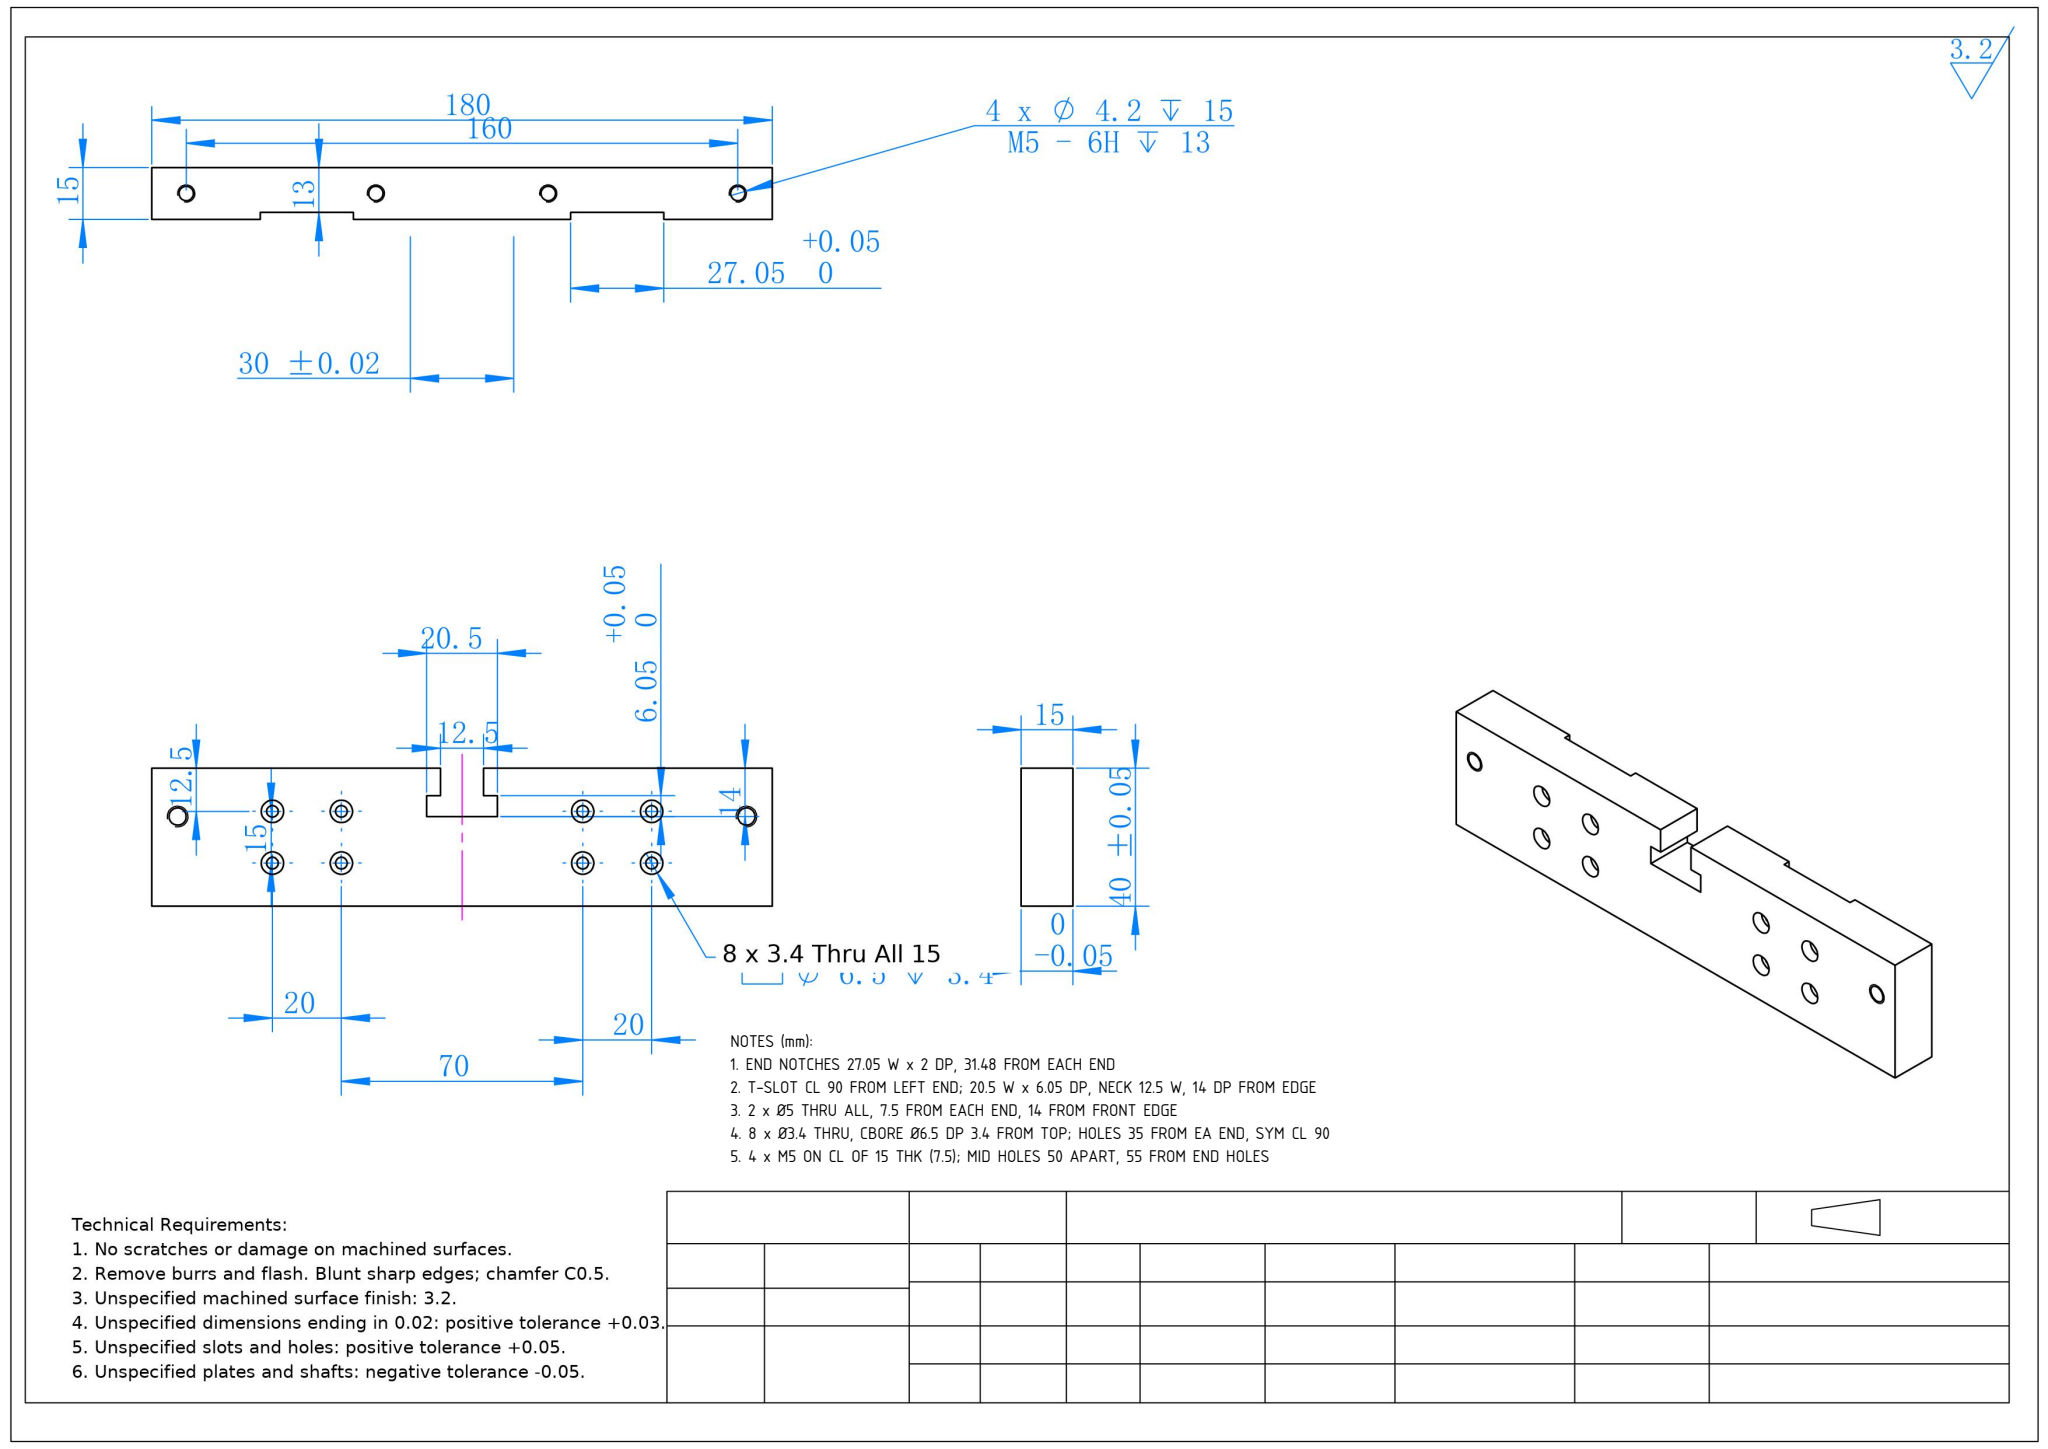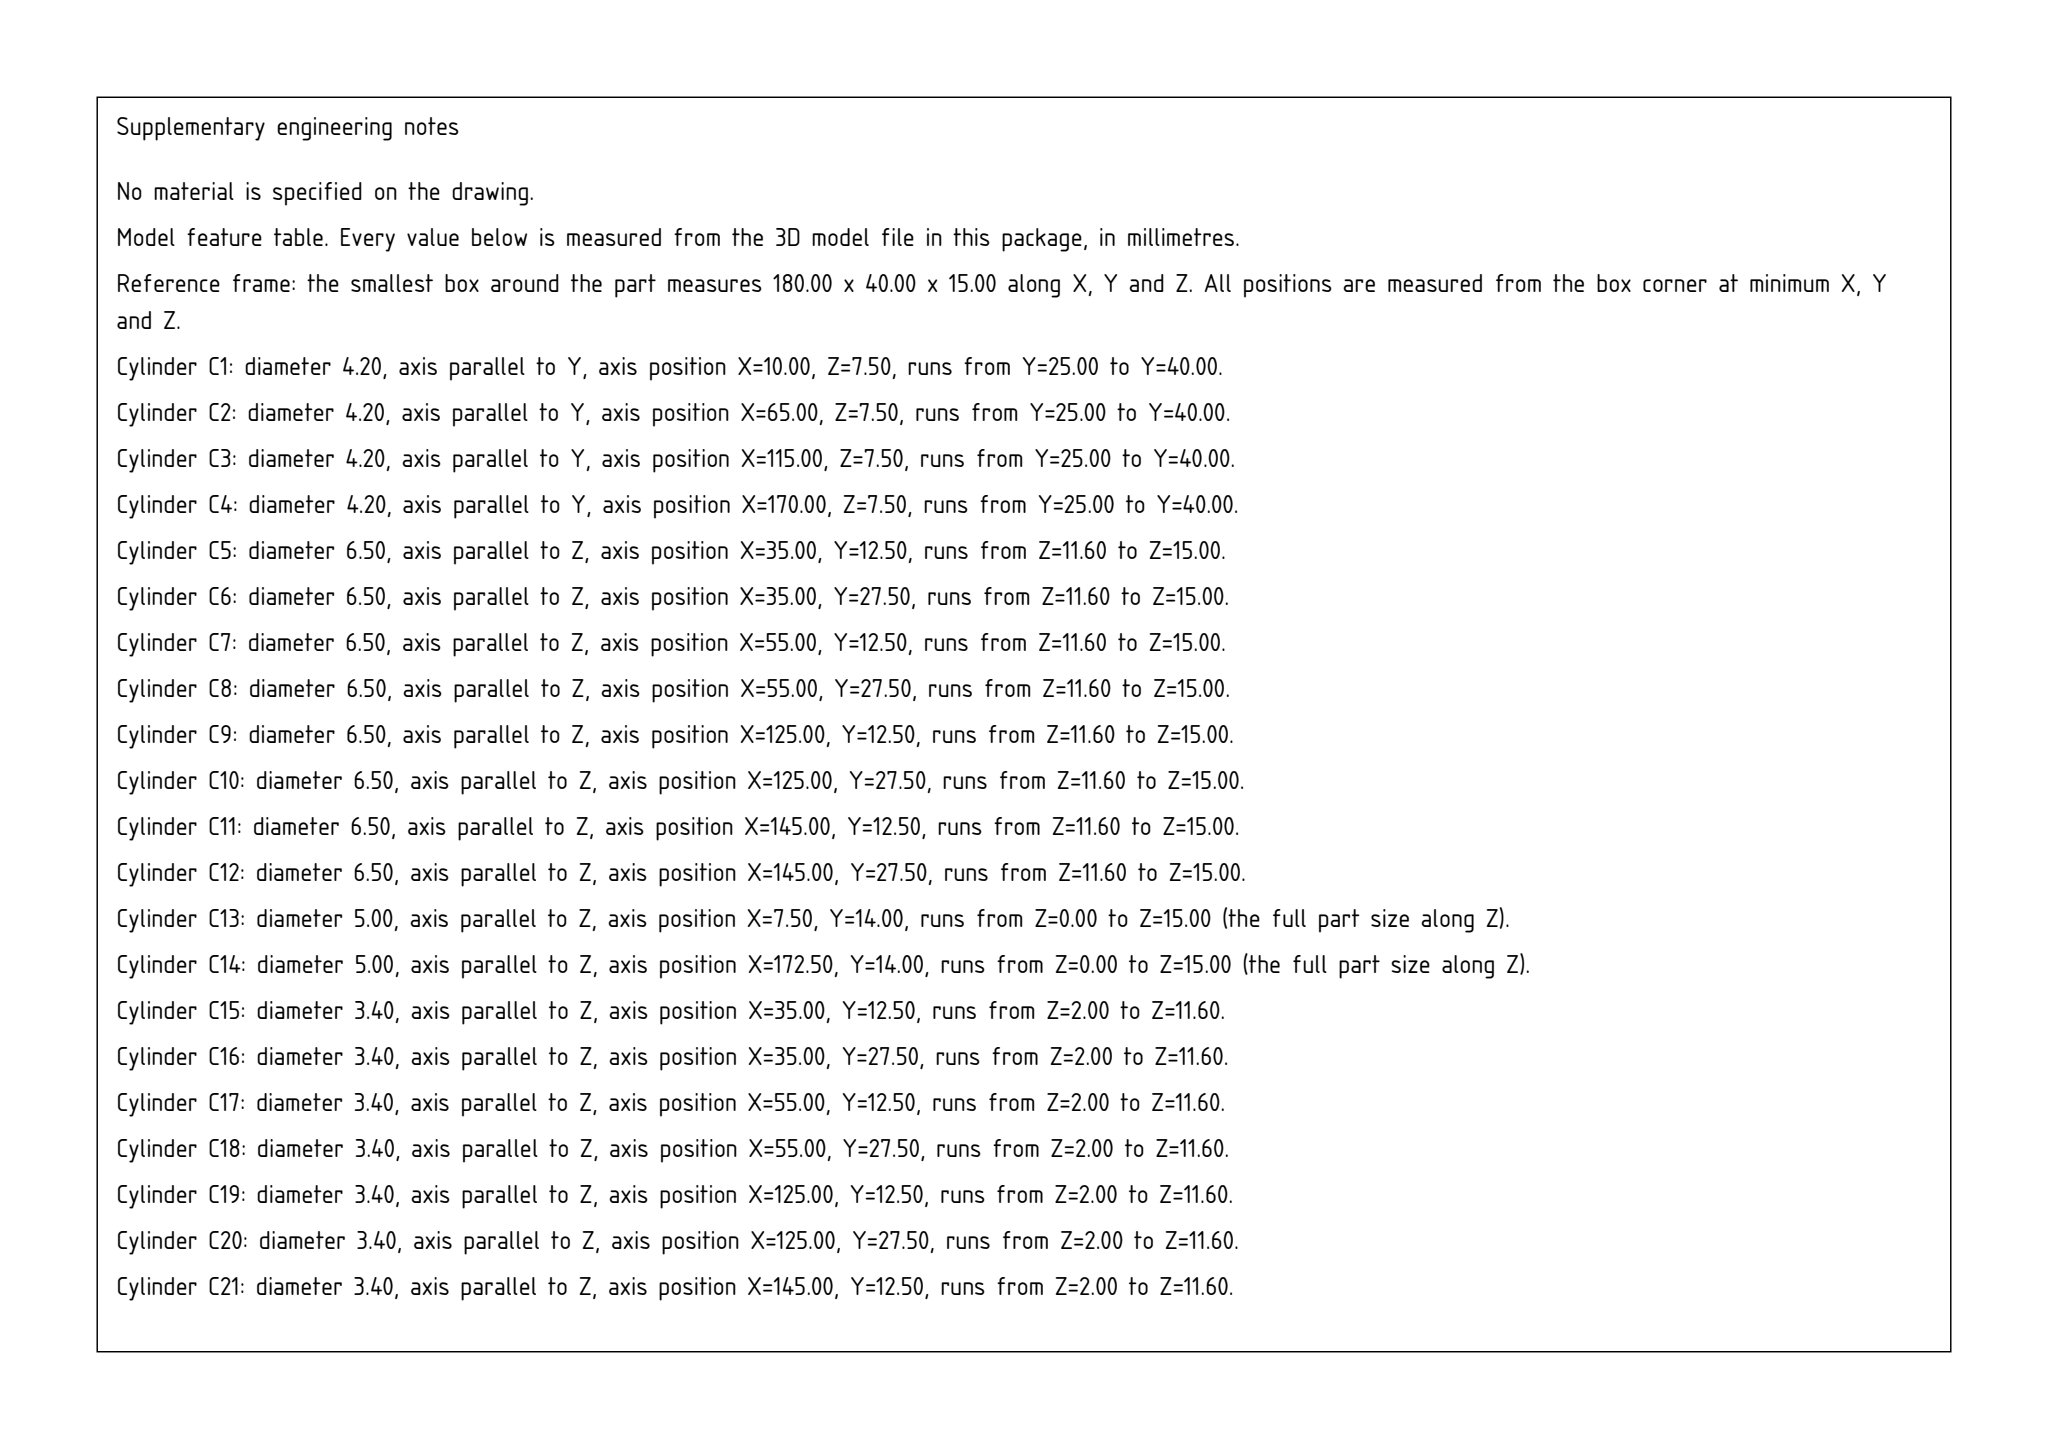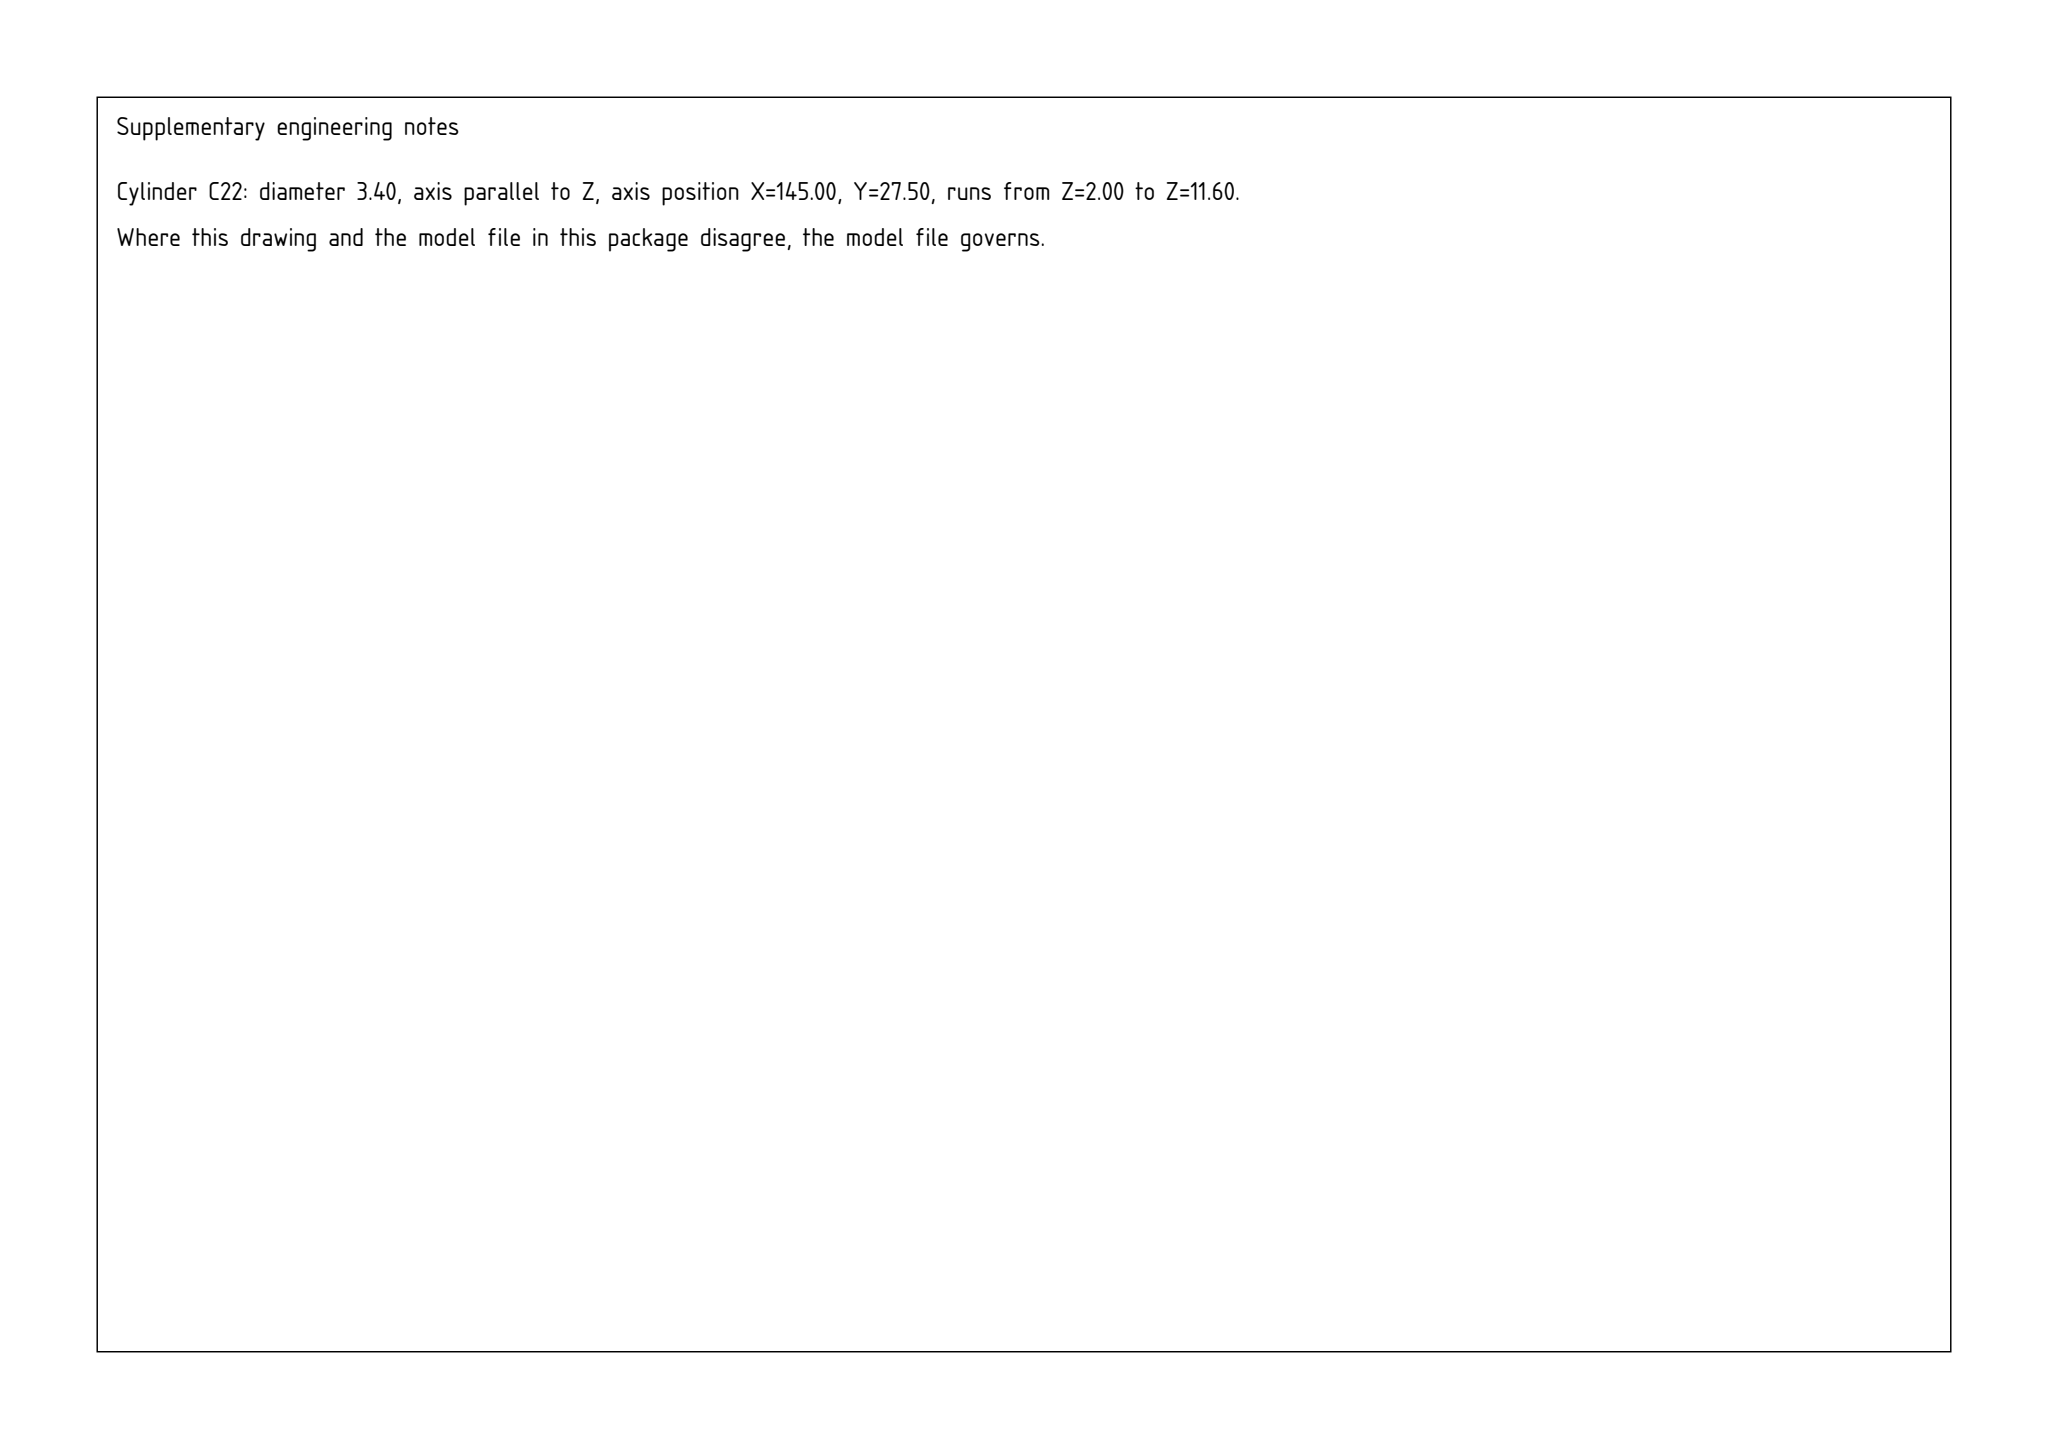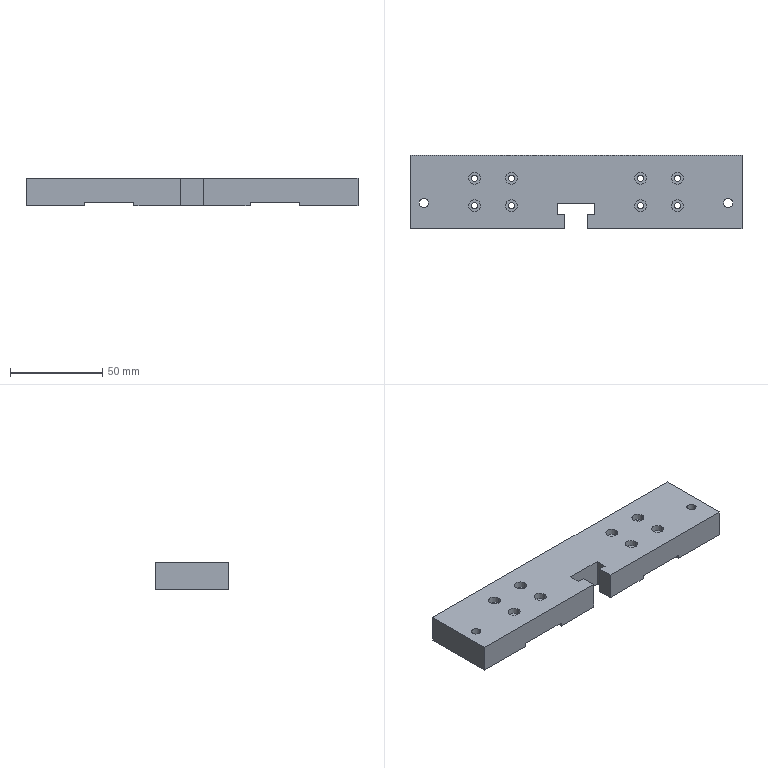Part | SolidWorks | mm | 1 solid | 82 faces | box 180 x 40 x 15 mm | volume 97278 mm3 | cylinder 44 | plane 30 | cone 8 | commonest cylinder face diameters 6.5 x16 3.4 x16 4.2 x8 5 x4
Drawing notes:
END NOTCHES 27.05 W x 2 DP, 31.48 FROM EACH END | from the solid: x planes 31.48/58.53 & 121.48/148.53; z plane 2.0
T-SLOT CL 90 FROM LEFT END; 20.5 W x 6.05 DP, NECK 12.5 W, 14 DP FROM EDGE | from the solid: x 79.75/100.25 = 20.5, x 83.75/96.25 = 12.5, mid 90; y planes 7.95 & 14.0
2 x Ø5 THRU ALL, 7.5 FROM EACH END, 14 FROM FRONT EDGE | from the solid: dia 5.0 axis z L15.0 at [7.5,14] and [172.5,14]; bbox X=180
8 x Ø3.4 THRU, CBORE Ø6.5 DP 3.4 FROM TOP; HOLES 35 FROM EA END, SYM CL 90 | from the solid: Ø3.4 L9.6 + coaxial Ø6.5 L3.4 at x=35,55,125,145; z plane 11.6 = 15-3.4
4 x M5 ON CL OF 15 THK (7.5); MID HOLES 50 APART, 55 FROM END HOLES | from the solid: Ø4.2 y-axis holes at x=10,65,115,170, z=7.5; 115-65=50, 65-10=55
build123d program:
from build123d import *

# Parameters (mm, degrees)
SKETCH1_W                                       = 180
SKETCH1_H                                       = 40
BOSS_EXTRUDE1_DEPTH                             = 15
CUT_EXTRUDE2_DEPTH                              = 94.408
SKETCH15_W                                      = 27.05
SKETCH15_H                                      = 40
CUT_EXTRUDE4_DEPTH                              = 2
M5_TAPPED_HOLE1_D                               = 4.2
M5_TAPPED_HOLE1_DEPTH                           = 15
M5_TAPPED_HOLE1_TIP                             = 1.262
M3_HEX_SOCKET_HEAD_CAP_SCREW_CBORE1_D           = 3.4
M3_HEX_SOCKET_HEAD_CAP_SCREW_CBORE1_CBORE_D     = 6.5
M3_HEX_SOCKET_HEAD_CAP_SCREW_CBORE1_CBORE_DEPTH = 3.4
M6_TAPPED_HOLE1_D                               = 5


with BuildPart() as part:
    # Sketch1 → Boss-Extrude1 (new body)
    with BuildSketch(Plane.XY):
        Rectangle(SKETCH1_W, SKETCH1_H)
    extrude(amount=BOSS_EXTRUDE1_DEPTH)

    # Sketch5 → Cut-Extrude2 (cut, through all)
    with BuildSketch(Plane.XY.offset(15)):
        Polygon((6.25, -12.05), (10.25, -12.05), (10.25, -6), (-10.25, -6), (-10.25, -12.05), (-6.25, -12.05), (-6.25, -20), (6.25, -20), align=None)
    extrude(amount=-CUT_EXTRUDE2_DEPTH, mode=Mode.SUBTRACT)

    # Sketch15 → Cut-Extrude4 (cut)
    with BuildSketch(Plane(origin=(0, 0, 0), x_dir=(-1, 0, 0), z_dir=(0, 0, -1))):
        with Locations((-45, 0)):
            Rectangle(SKETCH15_W, SKETCH15_H)
        with Locations((45, 0)):
            Rectangle(SKETCH15_W, SKETCH15_H)
    extrude(amount=-CUT_EXTRUDE4_DEPTH, mode=Mode.SUBTRACT)

    # M5 Tapped Hole1
    with Locations(Plane(origin=(0, 20, 0), x_dir=(-1, 0, 0), z_dir=(0, 1, 0))):
        with Locations((80, 7.5), (25, 7.5), (-80, 7.5), (-25, 7.5)):
            Hole(M5_TAPPED_HOLE1_D / 2, depth=M5_TAPPED_HOLE1_DEPTH)
            with Locations((0, 0, -(M5_TAPPED_HOLE1_DEPTH + M5_TAPPED_HOLE1_TIP / 2))):  # 118° drill point
                Cone(0, M5_TAPPED_HOLE1_D / 2, M5_TAPPED_HOLE1_TIP, mode=Mode.SUBTRACT)

    # M3 Hex Socket Head Cap Screw CBORE1 (through all)
    with Locations(Plane.XY.offset(15)):
        with Locations((35, 7.5), (35, -7.5), (55, 7.5), (55, -7.5), (-55, -7.5), (-55, 7.5), (-35, -7.5), (-35, 7.5)):
            CounterBoreHole(M3_HEX_SOCKET_HEAD_CAP_SCREW_CBORE1_D / 2, M3_HEX_SOCKET_HEAD_CAP_SCREW_CBORE1_CBORE_D / 2, M3_HEX_SOCKET_HEAD_CAP_SCREW_CBORE1_CBORE_DEPTH)

    # M6 Tapped Hole1 (through all)
    with Locations(Plane.XY.offset(15)):
        with Locations((82.5, -6), (-82.5, -6)):
            Hole(M6_TAPPED_HOLE1_D / 2)


solid = part.part